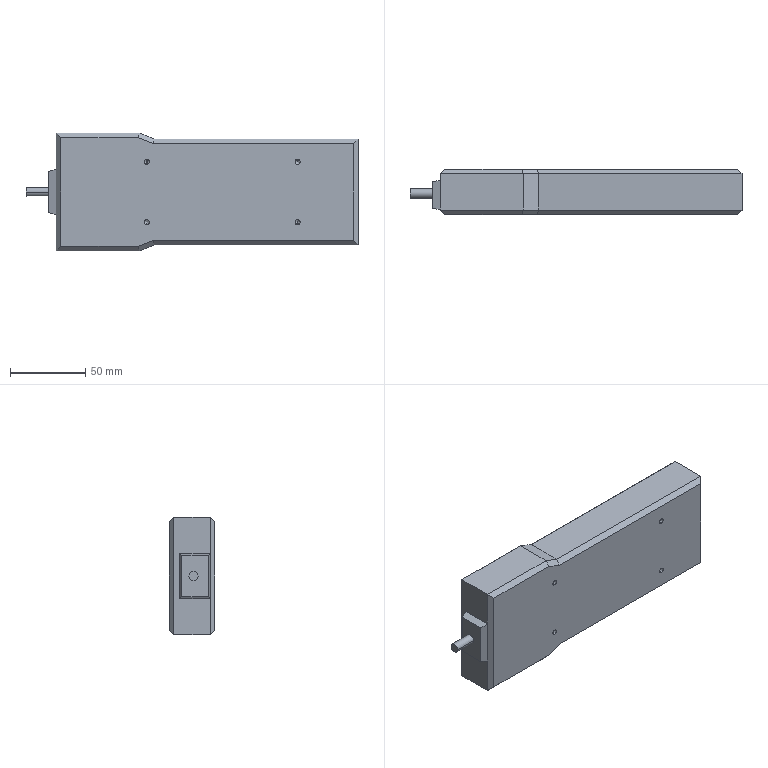Component | SolidWorks | CS021-DigitalPush-PullForceGaugeSF-500-2 | 1 solid | 51 faces | box 220 x 30 x 78 mm | volume 432270 mm3 | plane 33 | cylinder 10 | cone 8 | commonest cylinder face diameters 3.3 x8 6 x2 | material POM (White)
build123d program:
from build123d import *

# Parameters (mm, degrees)
BOSS_EXTRUDE1_DEPTH   = 15
CHAMFER1_SIZE         = 3
M4_TAPPED_HOLE1_D     = 3.3
M4_TAPPED_HOLE1_DEPTH = 10.1
M4_TAPPED_HOLE1_TIP   = 0.9914
SKETCH6_W             = 30
SKETCH6_H             = 20
BOSS_EXTRUDE3_DEPTH   = 5
BOSS_EXTRUDE3_TAPER   = 15
SKETCH5_R             = 3
BOSS_EXTRUDE2_DEPTH   = 15


with BuildPart() as part:
    # Sketch1 → Boss-Extrude1 (new, symmetric)
    with BuildSketch(Plane.XY):
        Polygon((-39, 200), (39, 200), (39, 145), (35, 135), (35, 0), (-35, 0), (-35, 135), (-39, 145), align=None)
    extrude(amount=BOSS_EXTRUDE1_DEPTH, both=True)

    # Chamfer1
    chamfer1_edges = [part.edges().sort_by_distance(p)[0] for p in [
        (-39, 172.5, 15),
        (0, 200, -15),
        (39, 172.5, -15),
        (-37, 140, 15),
        (-35, 67.5, 15),
        (0, 0, 15),
        (35, 67.5, 15),
        (37, 140, 15),
        (39, 172.5, 15),
        (0, 200, 15),
        (37, 140, -15),
        (35, 67.5, -15),
        (0, 0, -15),
        (-35, 67.5, -15),
        (-37, 140, -15),
        (-39, 172.5, -15),
    ]]
    chamfer(chamfer1_edges, length=CHAMFER1_SIZE)

    # M4 Tapped Hole1
    with Locations(Plane(origin=(0, 0, -15), x_dir=(-1, 0, 0), z_dir=(0, 0, -1))):
        with Locations((-20, 140), (-20, 40), (20, 40), (20, 140)):
            Hole(M4_TAPPED_HOLE1_D / 2, depth=M4_TAPPED_HOLE1_DEPTH)
            with Locations((0, 0, -(M4_TAPPED_HOLE1_DEPTH + M4_TAPPED_HOLE1_TIP / 2))):  # 118° drill point
                Cone(0, M4_TAPPED_HOLE1_D / 2, M4_TAPPED_HOLE1_TIP, mode=Mode.SUBTRACT)

    # Sketch6 → Boss-Extrude3 (add)
    with BuildSketch(Plane(origin=(0, 200, 0), x_dir=(1, 0, 0), z_dir=(0, 1, 0))):
        with Locations((0, 2)):
            Rectangle(SKETCH6_W, SKETCH6_H)
    extrude(amount=BOSS_EXTRUDE3_DEPTH, taper=BOSS_EXTRUDE3_TAPER)

    # Sketch5 → Boss-Extrude2 (add)
    with BuildSketch(Plane(origin=(0, 205, 0), x_dir=(1, 0, 0), z_dir=(0, 1, 0))):
        with Locations(Location((0, 1, 0), (0, 0, 270))):
            Circle(SKETCH5_R)
    extrude(amount=BOSS_EXTRUDE2_DEPTH)


solid = part.part

# Placed as in the assembly
solid = solid.moved(Location((237.448, 173.317, 0), (-90, 0, 90)))